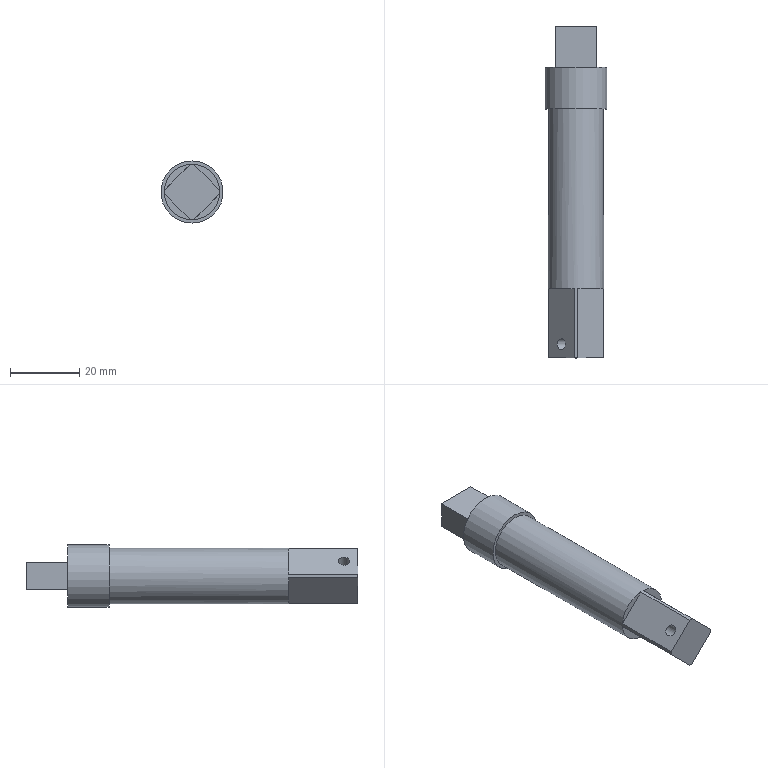Component | NX | VALVE_STEM | 1 solid | 19 faces | volume 17419 mm3 | plane 16 | cylinder 3 | commonest cylinder face diameters 16 x1 18 x1 3.3 x1